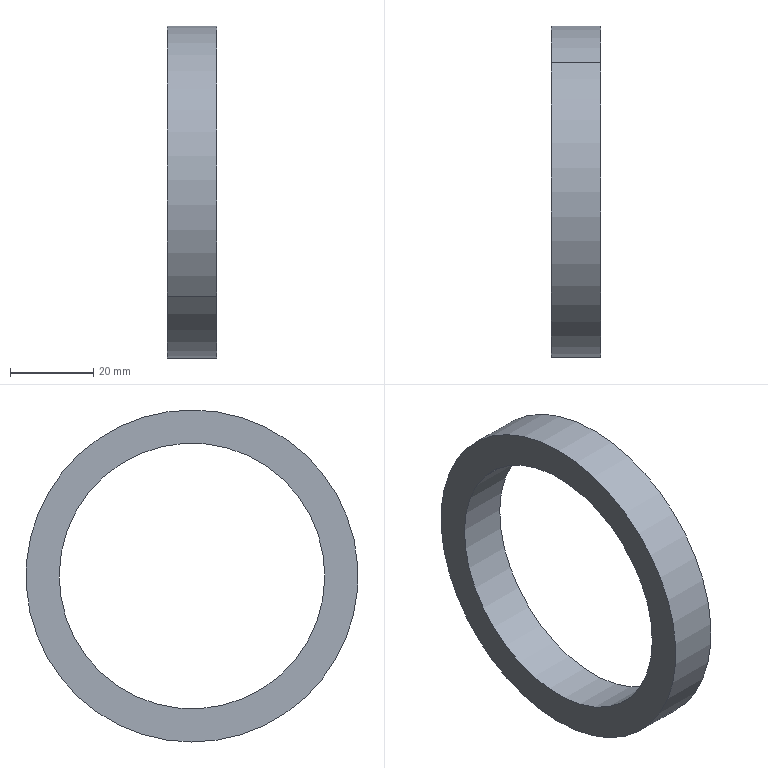Component | SolidWorks | 4-12-12ClampingAxisAssembly-1_4-12-11TelescopicAxisOilSealTC64X80X12-1 | 1 solid | 12 faces | box 12 x 80 x 80 mm | volume 18096 mm3 | cylinder 8 | plane 4 | commonest cylinder face diameters 68 x2 76 x2 64 x2 80 x2 | material Rubber
build123d program:
from build123d import *

# Parameters (mm, degrees)
SKETCH1_R          = 40
SKETCH1_R_2        = 32
EXTRUDE1_DEPTH     = 12
SKETCH2_R          = 38
SKETCH2_R_2        = 34
CUT_EXTRUDE1_DEPTH = 4


with BuildPart() as part:
    # Sketch1 → Extrude1 (new body)
    with BuildSketch(Plane(origin=(0, 0, 0), x_dir=(1, 0, 0), z_dir=(0, 1, 0))):
        with Locations(Location((0, 0, 0), (0, 0, 270))):
            Circle(SKETCH1_R)
        with Locations(Location((0, 0, 0), (0, 0, 270))):
            Circle(SKETCH1_R_2, mode=Mode.SUBTRACT)
    extrude(amount=EXTRUDE1_DEPTH)

    # Sketch2 → Cut-Extrude1 (cut)
    with BuildSketch(Plane(origin=(0, 12, 0), x_dir=(1, 0, 0), z_dir=(0, 1, 0))):
        with Locations(Location((0, 0, 0), (0, 0, 270))):
            Circle(SKETCH2_R)
        with Locations(Location((0, 0, 0), (0, 0, 270))):
            Circle(SKETCH2_R_2, mode=Mode.SUBTRACT)
    extrude(amount=-CUT_EXTRUDE1_DEPTH, mode=Mode.SUBTRACT)


solid = part.part

# Placed as in the assembly
solid = solid.moved(Location((-87.809, -4.181, 0), (0, 0, -90)))
STEP:
#1=COLOUR_RGB('',0.7922,0.8196,0.9333);
#2=FILL_AREA_STYLE_COLOUR('',#1);
#3=FILL_AREA_STYLE('',(#2));
#4=SURFACE_STYLE_FILL_AREA(#3);
#5=SURFACE_SIDE_STYLE('',(#4));
#6=SURFACE_STYLE_USAGE(.BOTH.,#5);
#7=PRESENTATION_STYLE_ASSIGNMENT((#6));
#8=CARTESIAN_POINT('',(-3.142,0.8782,0.8392));
#9=VERTEX_POINT('',#8);
#10=CARTESIAN_POINT('',(-3.142,-1.207,-0.8392));
#11=VERTEX_POINT('',#10);
#12=CARTESIAN_POINT('',(-3.142,-0.1646,0.));
#13=DIRECTION('',(1.,0.,-0.));
#14=DIRECTION('',(0.,0.7791,0.6269));
#15=AXIS2_PLACEMENT_3D('',#12,#13,#14);
#16=CIRCLE('',#15,1.339);
#17=EDGE_CURVE('',#9,#11,#16,.T.);
#18=ORIENTED_EDGE('',*,*,#17,.T.);
#19=CARTESIAN_POINT('',(-2.985,-1.207,-0.8392));
#20=VERTEX_POINT('',#19);
#21=CARTESIAN_POINT('',(-3.142,-1.207,-0.8392));
#22=DIRECTION('',(1.,0.,-0.));
#23=VECTOR('',#22,39.37);
#24=LINE('',#21,#23);
#25=EDGE_CURVE('',#11,#20,#24,.T.);
#26=ORIENTED_EDGE('',*,*,#25,.T.);
#27=CARTESIAN_POINT('',(-2.985,0.8782,0.8392));
#28=VERTEX_POINT('',#27);
#29=CARTESIAN_POINT('',(-2.985,-0.1646,0.));
#30=DIRECTION('',(1.,0.,-0.));
#31=DIRECTION('',(0.,0.7791,0.6269));
#32=AXIS2_PLACEMENT_3D('',#29,#30,#31);
#33=CIRCLE('',#32,1.339);
#34=EDGE_CURVE('',#28,#20,#33,.T.);
#35=ORIENTED_EDGE('',*,*,#34,.F.);
#36=CARTESIAN_POINT('',(-3.142,0.8782,0.8392));
#37=DIRECTION('',(1.,0.,-0.));
#38=VECTOR('',#37,39.37);
#39=LINE('',#36,#38);
#40=EDGE_CURVE('',#9,#28,#39,.T.);
#41=ORIENTED_EDGE('',*,*,#40,.F.);
#42=EDGE_LOOP('',(#18,#26,#35,#41));
#43=FACE_OUTER_BOUND('',#42,.T.);
#44=CARTESIAN_POINT('',(-3.142,-0.1646,0.));
#45=DIRECTION('',(1.,0.,-0.));
#46=DIRECTION('',(0.,0.7791,0.6269));
#47=AXIS2_PLACEMENT_3D('',#44,#45,#46);
#48=CYLINDRICAL_SURFACE('',#47,1.339);
#49=ADVANCED_FACE('',(#43),#48,.T.);
#50=CARTESIAN_POINT('',(-3.142,-1.33,-0.938));
#51=VERTEX_POINT('',#50);
#52=CARTESIAN_POINT('',(-3.142,1.001,0.938));
#53=VERTEX_POINT('',#52);
#54=CARTESIAN_POINT('',(-3.142,-0.1646,0.));
#55=DIRECTION('',(1.,0.,-0.));
#56=DIRECTION('',(0.,0.7791,0.6269));
#57=AXIS2_PLACEMENT_3D('',#54,#55,#56);
#58=CIRCLE('',#57,1.496);
#59=EDGE_CURVE('',#51,#53,#58,.T.);
#60=ORIENTED_EDGE('',*,*,#59,.F.);
#61=CARTESIAN_POINT('',(-2.985,-1.33,-0.938));
#62=VERTEX_POINT('',#61);
#63=CARTESIAN_POINT('',(-3.142,-1.33,-0.938));
#64=DIRECTION('',(1.,0.,-0.));
#65=VECTOR('',#64,39.37);
#66=LINE('',#63,#65);
#67=EDGE_CURVE('',#51,#62,#66,.T.);
#68=ORIENTED_EDGE('',*,*,#67,.T.);
#69=CARTESIAN_POINT('',(-2.985,1.001,0.938));
#70=VERTEX_POINT('',#69);
#71=CARTESIAN_POINT('',(-2.985,-0.1646,0.));
#72=DIRECTION('',(1.,0.,-0.));
#73=DIRECTION('',(0.,0.7791,0.6269));
#74=AXIS2_PLACEMENT_3D('',#71,#72,#73);
#75=CIRCLE('',#74,1.496);
#76=EDGE_CURVE('',#62,#70,#75,.T.);
#77=ORIENTED_EDGE('',*,*,#76,.T.);
#78=CARTESIAN_POINT('',(-3.142,1.001,0.938));
#79=DIRECTION('',(1.,0.,-0.));
#80=VECTOR('',#79,39.37);
#81=LINE('',#78,#80);
#82=EDGE_CURVE('',#53,#70,#81,.T.);
#83=ORIENTED_EDGE('',*,*,#82,.F.);
#84=EDGE_LOOP('',(#60,#68,#77,#83));
#85=FACE_OUTER_BOUND('',#84,.T.);
#86=CARTESIAN_POINT('',(-3.142,-0.1646,0.));
#87=DIRECTION('',(1.,0.,-0.));
#88=DIRECTION('',(0.,0.7791,0.6269));
#89=AXIS2_PLACEMENT_3D('',#86,#87,#88);
#90=CYLINDRICAL_SURFACE('',#89,1.496);
#91=ADVANCED_FACE('',(#85),#90,.F.);
#92=CARTESIAN_POINT('',(-2.985,-1.146,-0.7899));
#93=VERTEX_POINT('',#92);
#94=CARTESIAN_POINT('',(-2.985,0.8169,0.7899));
#95=VERTEX_POINT('',#94);
#96=CARTESIAN_POINT('',(-2.985,-0.1646,0.));
#97=DIRECTION('',(1.,0.,-0.));
#98=DIRECTION('',(0.,0.7791,0.6269));
#99=AXIS2_PLACEMENT_3D('',#96,#97,#98);
#100=CIRCLE('',#99,1.26);
#101=EDGE_CURVE('',#93,#95,#100,.T.);
#102=ORIENTED_EDGE('',*,*,#101,.T.);
#103=CARTESIAN_POINT('',(-3.457,0.8169,0.7899));
#104=VERTEX_POINT('',#103);
#105=CARTESIAN_POINT('',(-2.985,0.8169,0.7899));
#106=DIRECTION('',(-1.,-0.,0.));
#107=VECTOR('',#106,39.37);
#108=LINE('',#105,#107);
#109=EDGE_CURVE('',#95,#104,#108,.T.);
#110=ORIENTED_EDGE('',*,*,#109,.T.);
#111=CARTESIAN_POINT('',(-3.457,-1.146,-0.7899));
#112=VERTEX_POINT('',#111);
#113=CARTESIAN_POINT('',(-3.457,-0.1646,0.));
#114=DIRECTION('',(1.,0.,-0.));
#115=DIRECTION('',(0.,0.7791,0.6269));
#116=AXIS2_PLACEMENT_3D('',#113,#114,#115);
#117=CIRCLE('',#116,1.26);
#118=EDGE_CURVE('',#112,#104,#117,.T.);
#119=ORIENTED_EDGE('',*,*,#118,.F.);
#120=CARTESIAN_POINT('',(-2.985,-1.146,-0.7899));
#121=DIRECTION('',(-1.,-0.,0.));
#122=VECTOR('',#121,39.37);
#123=LINE('',#120,#122);
#124=EDGE_CURVE('',#93,#112,#123,.T.);
#125=ORIENTED_EDGE('',*,*,#124,.F.);
#126=EDGE_LOOP('',(#102,#110,#119,#125));
#127=FACE_OUTER_BOUND('',#126,.T.);
#128=CARTESIAN_POINT('',(-2.985,-0.1646,0.));
#129=DIRECTION('',(-1.,-0.,0.));
#130=DIRECTION('',(0.,-0.7791,-0.6269));
#131=AXIS2_PLACEMENT_3D('',#128,#129,#130);
#132=CYLINDRICAL_SURFACE('',#131,1.26);
#133=ADVANCED_FACE('',(#127),#132,.F.);
#134=CARTESIAN_POINT('',(-2.985,1.062,0.9873));
#135=VERTEX_POINT('',#134);
#136=CARTESIAN_POINT('',(-2.985,-1.391,-0.9873));
#137=VERTEX_POINT('',#136);
#138=CARTESIAN_POINT('',(-2.985,-0.1646,0.));
#139=DIRECTION('',(1.,0.,-0.));
#140=DIRECTION('',(0.,0.7791,0.6269));
#141=AXIS2_PLACEMENT_3D('',#138,#139,#140);
#142=CIRCLE('',#141,1.575);
#143=EDGE_CURVE('',#135,#137,#142,.T.);
#144=ORIENTED_EDGE('',*,*,#143,.F.);
#145=CARTESIAN_POINT('',(-3.457,1.062,0.9873));
#146=VERTEX_POINT('',#145);
#147=CARTESIAN_POINT('',(-2.985,1.062,0.9873));
#148=DIRECTION('',(-1.,-0.,0.));
#149=VECTOR('',#148,39.37);
#150=LINE('',#147,#149);
#151=EDGE_CURVE('',#135,#146,#150,.T.);
#152=ORIENTED_EDGE('',*,*,#151,.T.);
#153=CARTESIAN_POINT('',(-3.457,-1.391,-0.9873));
#154=VERTEX_POINT('',#153);
#155=CARTESIAN_POINT('',(-3.457,-0.1646,0.));
#156=DIRECTION('',(1.,0.,-0.));
#157=DIRECTION('',(0.,0.7791,0.6269));
#158=AXIS2_PLACEMENT_3D('',#155,#156,#157);
#159=CIRCLE('',#158,1.575);
#160=EDGE_CURVE('',#146,#154,#159,.T.);
#161=ORIENTED_EDGE('',*,*,#160,.T.);
#162=CARTESIAN_POINT('',(-2.985,-1.391,-0.9873));
#163=DIRECTION('',(-1.,-0.,0.));
#164=VECTOR('',#163,39.37);
#165=LINE('',#162,#164);
#166=EDGE_CURVE('',#137,#154,#165,.T.);
#167=ORIENTED_EDGE('',*,*,#166,.F.);
#168=EDGE_LOOP('',(#144,#152,#161,#167));
#169=FACE_OUTER_BOUND('',#168,.T.);
#170=CARTESIAN_POINT('',(-2.985,-0.1646,0.));
#171=DIRECTION('',(-1.,-0.,0.));
#172=DIRECTION('',(0.,-0.7791,-0.6269));
#173=AXIS2_PLACEMENT_3D('',#170,#171,#172);
#174=CYLINDRICAL_SURFACE('',#173,1.575);
#175=ADVANCED_FACE('',(#169),#174,.T.);
#176=ORIENTED_EDGE('',*,*,#101,.F.);
#177=CARTESIAN_POINT('',(-2.985,-0.1646,0.));
#178=DIRECTION('',(1.,0.,-0.));
#179=DIRECTION('',(0.,0.7791,0.6269));
#180=AXIS2_PLACEMENT_3D('',#177,#178,#179);
#181=CIRCLE('',#180,1.26);
#182=EDGE_CURVE('',#95,#93,#181,.T.);
#183=ORIENTED_EDGE('',*,*,#182,.F.);
#184=EDGE_LOOP('',(#176,#183));
#185=FACE_BOUND('',#184,.T.);
#186=ORIENTED_EDGE('',*,*,#34,.T.);
#187=CARTESIAN_POINT('',(-2.985,-0.1646,0.));
#188=DIRECTION('',(1.,0.,-0.));
#189=DIRECTION('',(0.,0.7791,0.6269));
#190=AXIS2_PLACEMENT_3D('',#187,#188,#189);
#191=CIRCLE('',#190,1.339);
#192=EDGE_CURVE('',#20,#28,#191,.T.);
#193=ORIENTED_EDGE('',*,*,#192,.T.);
#194=EDGE_LOOP('',(#186,#193));
#195=FACE_OUTER_BOUND('',#194,.T.);
#196=CARTESIAN_POINT('',(-2.985,-0.1646,0.));
#197=DIRECTION('',(1.,0.,-0.));
#198=DIRECTION('',(-0.,0.7791,0.6269));
#199=AXIS2_PLACEMENT_3D('',#196,#197,#198);
#200=PLANE('',#199);
#201=ADVANCED_FACE('',(#185,#195),#200,.T.);
#202=CARTESIAN_POINT('',(-2.985,-0.1646,0.));
#203=DIRECTION('',(1.,0.,-0.));
#204=DIRECTION('',(0.,0.7791,0.6269));
#205=AXIS2_PLACEMENT_3D('',#202,#203,#204);
#206=CIRCLE('',#205,1.496);
#207=EDGE_CURVE('',#70,#62,#206,.T.);
#208=ORIENTED_EDGE('',*,*,#207,.F.);
#209=ORIENTED_EDGE('',*,*,#76,.F.);
#210=EDGE_LOOP('',(#208,#209));
#211=FACE_BOUND('',#210,.T.);
#212=CARTESIAN_POINT('',(-2.985,-0.1646,0.));
#213=DIRECTION('',(1.,0.,-0.));
#214=DIRECTION('',(0.,0.7791,0.6269));
#215=AXIS2_PLACEMENT_3D('',#212,#213,#214);
#216=CIRCLE('',#215,1.575);
#217=EDGE_CURVE('',#137,#135,#216,.T.);
#218=ORIENTED_EDGE('',*,*,#217,.T.);
#219=ORIENTED_EDGE('',*,*,#143,.T.);
#220=EDGE_LOOP('',(#218,#219));
#221=FACE_OUTER_BOUND('',#220,.T.);
#222=CARTESIAN_POINT('',(-2.985,-0.1646,0.));
#223=DIRECTION('',(1.,0.,-0.));
#224=DIRECTION('',(-0.,0.7791,0.6269));
#225=AXIS2_PLACEMENT_3D('',#222,#223,#224);
#226=PLANE('',#225);
#227=ADVANCED_FACE('',(#211,#221),#226,.T.);
#228=CARTESIAN_POINT('',(-3.457,-0.1646,0.));
#229=DIRECTION('',(1.,0.,-0.));
#230=DIRECTION('',(0.,0.7791,0.6269));
#231=AXIS2_PLACEMENT_3D('',#228,#229,#230);
#232=CIRCLE('',#231,1.575);
#233=EDGE_CURVE('',#154,#146,#232,.T.);
#234=ORIENTED_EDGE('',*,*,#233,.F.);
#235=ORIENTED_EDGE('',*,*,#160,.F.);
#236=EDGE_LOOP('',(#234,#235));
#237=FACE_OUTER_BOUND('',#236,.T.);
#238=ORIENTED_EDGE('',*,*,#118,.T.);
#239=CARTESIAN_POINT('',(-3.457,-0.1646,0.));
#240=DIRECTION('',(1.,0.,-0.));
#241=DIRECTION('',(0.,0.7791,0.6269));
#242=AXIS2_PLACEMENT_3D('',#239,#240,#241);
#243=CIRCLE('',#242,1.26);
#244=EDGE_CURVE('',#104,#112,#243,.T.);
#245=ORIENTED_EDGE('',*,*,#244,.T.);
#246=EDGE_LOOP('',(#238,#245));
#247=FACE_BOUND('',#246,.T.);
#248=CARTESIAN_POINT('',(-3.457,-0.1646,0.));
#249=DIRECTION('',(1.,0.,-0.));
#250=DIRECTION('',(-0.,0.7791,0.6269));
#251=AXIS2_PLACEMENT_3D('',#248,#249,#250);
#252=PLANE('',#251);
#253=ADVANCED_FACE('',(#237,#247),#252,.F.);
#254=ORIENTED_EDGE('',*,*,#151,.F.);
#255=ORIENTED_EDGE('',*,*,#217,.F.);
#256=ORIENTED_EDGE('',*,*,#166,.T.);
#257=ORIENTED_EDGE('',*,*,#233,.T.);
#258=EDGE_LOOP('',(#254,#255,#256,#257));
#259=FACE_OUTER_BOUND('',#258,.T.);
#260=CARTESIAN_POINT('',(-2.985,-0.1646,0.));
#261=DIRECTION('',(-1.,-0.,0.));
#262=DIRECTION('',(0.,-0.7791,-0.6269));
#263=AXIS2_PLACEMENT_3D('',#260,#261,#262);
#264=CYLINDRICAL_SURFACE('',#263,1.575);
#265=ADVANCED_FACE('',(#259),#264,.T.);
#266=ORIENTED_EDGE('',*,*,#109,.F.);
#267=ORIENTED_EDGE('',*,*,#182,.T.);
#268=ORIENTED_EDGE('',*,*,#124,.T.);
#269=ORIENTED_EDGE('',*,*,#244,.F.);
#270=EDGE_LOOP('',(#266,#267,#268,#269));
#271=FACE_OUTER_BOUND('',#270,.T.);
#272=CARTESIAN_POINT('',(-2.985,-0.1646,0.));
#273=DIRECTION('',(-1.,-0.,0.));
#274=DIRECTION('',(0.,-0.7791,-0.6269));
#275=AXIS2_PLACEMENT_3D('',#272,#273,#274);
#276=CYLINDRICAL_SURFACE('',#275,1.26);
#277=ADVANCED_FACE('',(#271),#276,.F.);
#278=ORIENTED_EDGE('',*,*,#67,.F.);
#279=CARTESIAN_POINT('',(-3.142,-0.1646,0.));
#280=DIRECTION('',(1.,0.,-0.));
#281=DIRECTION('',(0.,0.7791,0.6269));
#282=AXIS2_PLACEMENT_3D('',#279,#280,#281);
#283=CIRCLE('',#282,1.496);
#284=EDGE_CURVE('',#53,#51,#283,.T.);
#285=ORIENTED_EDGE('',*,*,#284,.F.);
#286=ORIENTED_EDGE('',*,*,#82,.T.);
#287=ORIENTED_EDGE('',*,*,#207,.T.);
#288=EDGE_LOOP('',(#278,#285,#286,#287));
#289=FACE_OUTER_BOUND('',#288,.T.);
#290=CARTESIAN_POINT('',(-3.142,-0.1646,0.));
#291=DIRECTION('',(1.,0.,-0.));
#292=DIRECTION('',(0.,0.7791,0.6269));
#293=AXIS2_PLACEMENT_3D('',#290,#291,#292);
#294=CYLINDRICAL_SURFACE('',#293,1.496);
#295=ADVANCED_FACE('',(#289),#294,.F.);
#296=ORIENTED_EDGE('',*,*,#17,.F.);
#297=CARTESIAN_POINT('',(-3.142,-0.1646,0.));
#298=DIRECTION('',(1.,0.,-0.));
#299=DIRECTION('',(0.,0.7791,0.6269));
#300=AXIS2_PLACEMENT_3D('',#297,#298,#299);
#301=CIRCLE('',#300,1.339);
#302=EDGE_CURVE('',#11,#9,#301,.T.);
#303=ORIENTED_EDGE('',*,*,#302,.F.);
#304=EDGE_LOOP('',(#296,#303));
#305=FACE_BOUND('',#304,.T.);
#306=ORIENTED_EDGE('',*,*,#284,.T.);
#307=ORIENTED_EDGE('',*,*,#59,.T.);
#308=EDGE_LOOP('',(#306,#307));
#309=FACE_OUTER_BOUND('',#308,.T.);
#310=CARTESIAN_POINT('',(-3.142,-0.1646,0.));
#311=DIRECTION('',(1.,0.,-0.));
#312=DIRECTION('',(-0.,0.7791,0.6269));
#313=AXIS2_PLACEMENT_3D('',#310,#311,#312);
#314=PLANE('',#313);
#315=ADVANCED_FACE('',(#305,#309),#314,.T.);
#316=ORIENTED_EDGE('',*,*,#25,.F.);
#317=ORIENTED_EDGE('',*,*,#302,.T.);
#318=ORIENTED_EDGE('',*,*,#40,.T.);
#319=ORIENTED_EDGE('',*,*,#192,.F.);
#320=EDGE_LOOP('',(#316,#317,#318,#319));
#321=FACE_OUTER_BOUND('',#320,.T.);
#322=CARTESIAN_POINT('',(-3.142,-0.1646,0.));
#323=DIRECTION('',(1.,0.,-0.));
#324=DIRECTION('',(0.,0.7791,0.6269));
#325=AXIS2_PLACEMENT_3D('',#322,#323,#324);
#326=CYLINDRICAL_SURFACE('',#325,1.339);
#327=ADVANCED_FACE('',(#321),#326,.T.);
#328=CLOSED_SHELL('',(#49,#91,#133,#175,#201,#227,#253,#265,#277,#295,#315,#327));
#329=MANIFOLD_SOLID_BREP('',#328);
#330=STYLED_ITEM('',(#7),#329);
#331=(LENGTH_UNIT()NAMED_UNIT(*)SI_UNIT($,.METRE.));
#332=LENGTH_MEASURE_WITH_UNIT(LENGTH_MEASURE(0.0254),#331);
#333=DIMENSIONAL_EXPONENTS(1.,0.,0.,0.,0.,0.,0.);
#334=(CONVERSION_BASED_UNIT('',#332)LENGTH_UNIT()NAMED_UNIT(#333));
#335=UNCERTAINTY_MEASURE_WITH_UNIT(LENGTH_MEASURE(0.00001),#334,'','');
#336=(NAMED_UNIT(*)PLANE_ANGLE_UNIT()SI_UNIT($,.RADIAN.));
#337=(NAMED_UNIT(*)SI_UNIT($,.STERADIAN.)SOLID_ANGLE_UNIT());
#338=(GEOMETRIC_REPRESENTATION_CONTEXT(3)GLOBAL_UNCERTAINTY_ASSIGNED_CONTEXT((#335))GLOBAL_UNIT_ASSIGNED_CONTEXT((#334,#336,#337))REPRESENTATION_CONTEXT('',''));
#339=MECHANICAL_DESIGN_GEOMETRIC_PRESENTATION_REPRESENTATION('',(#330),#338);
#340=PRESENTATION_LAYER_ASSIGNMENT('','',(#330));
#341=CARTESIAN_POINT('',(0.,0.,0.));
#342=DIRECTION('',(0.,0.,1.));
#343=DIRECTION('',(1.,0.,0.));
#344=AXIS2_PLACEMENT_3D('',#341,#342,#343);
#345=(LENGTH_UNIT()NAMED_UNIT(*)SI_UNIT($,.METRE.));
#346=LENGTH_MEASURE_WITH_UNIT(LENGTH_MEASURE(0.0254),#345);
#347=DIMENSIONAL_EXPONENTS(1.,0.,0.,0.,0.,0.,0.);
#348=(CONVERSION_BASED_UNIT('',#346)LENGTH_UNIT()NAMED_UNIT(#347));
#349=UNCERTAINTY_MEASURE_WITH_UNIT(LENGTH_MEASURE(0.00001),#348,'','');
#350=(NAMED_UNIT(*)PLANE_ANGLE_UNIT()SI_UNIT($,.RADIAN.));
#351=(NAMED_UNIT(*)SI_UNIT($,.STERADIAN.)SOLID_ANGLE_UNIT());
#352=(GEOMETRIC_REPRESENTATION_CONTEXT(3)GLOBAL_UNCERTAINTY_ASSIGNED_CONTEXT((#349))GLOBAL_UNIT_ASSIGNED_CONTEXT((#348,#350,#351))REPRESENTATION_CONTEXT('',''));
#353=ADVANCED_BREP_SHAPE_REPRESENTATION('',(#329,#344),#352);